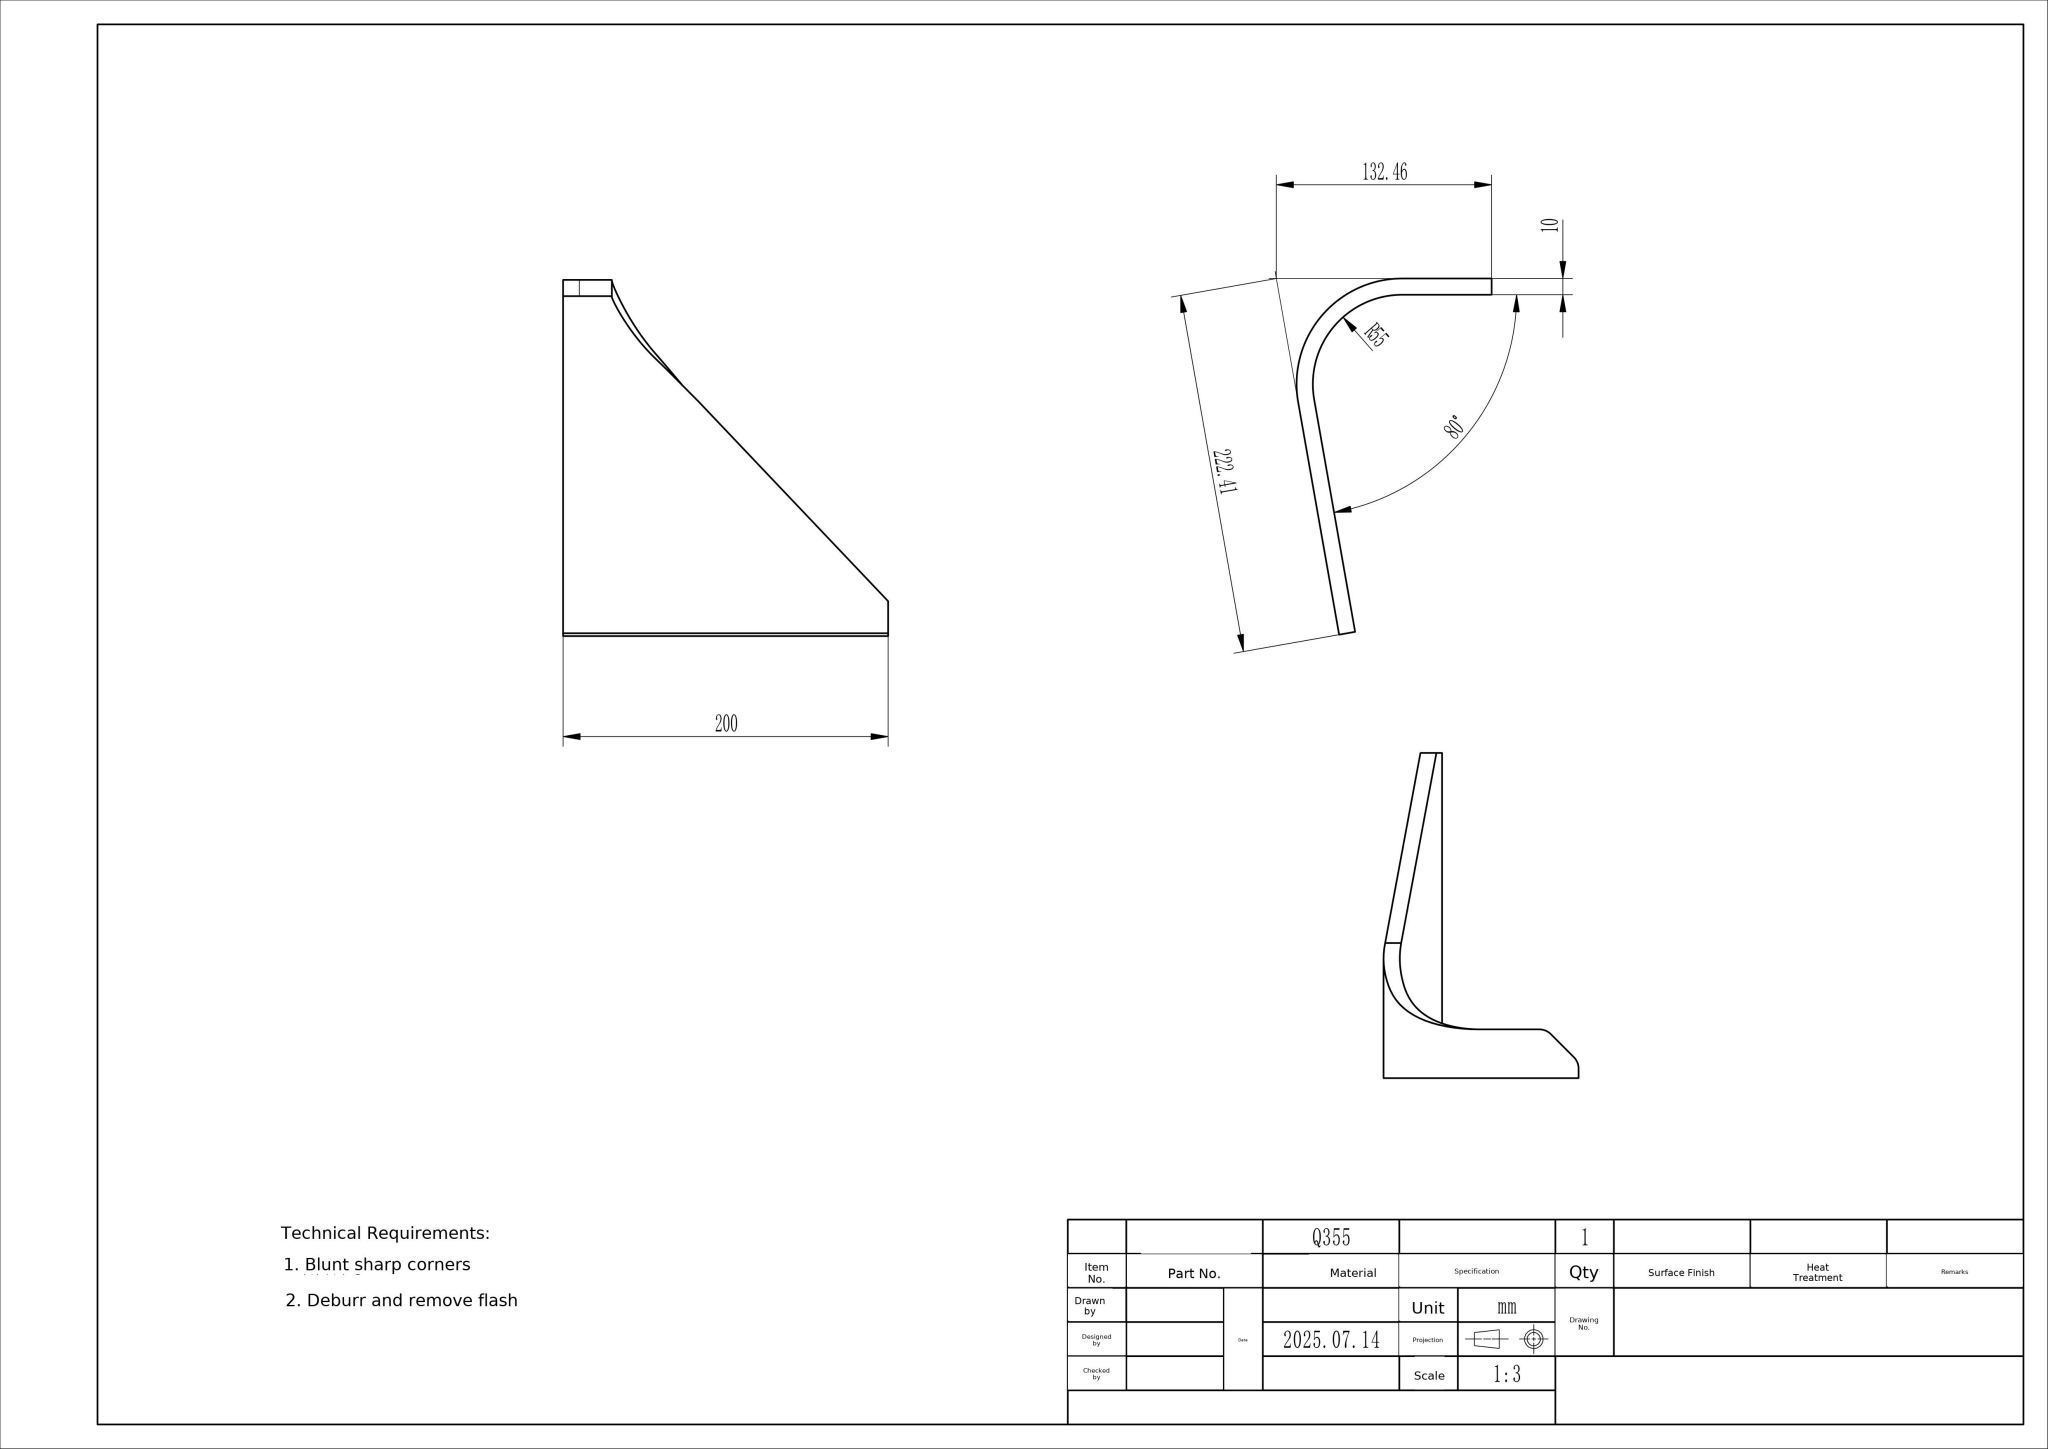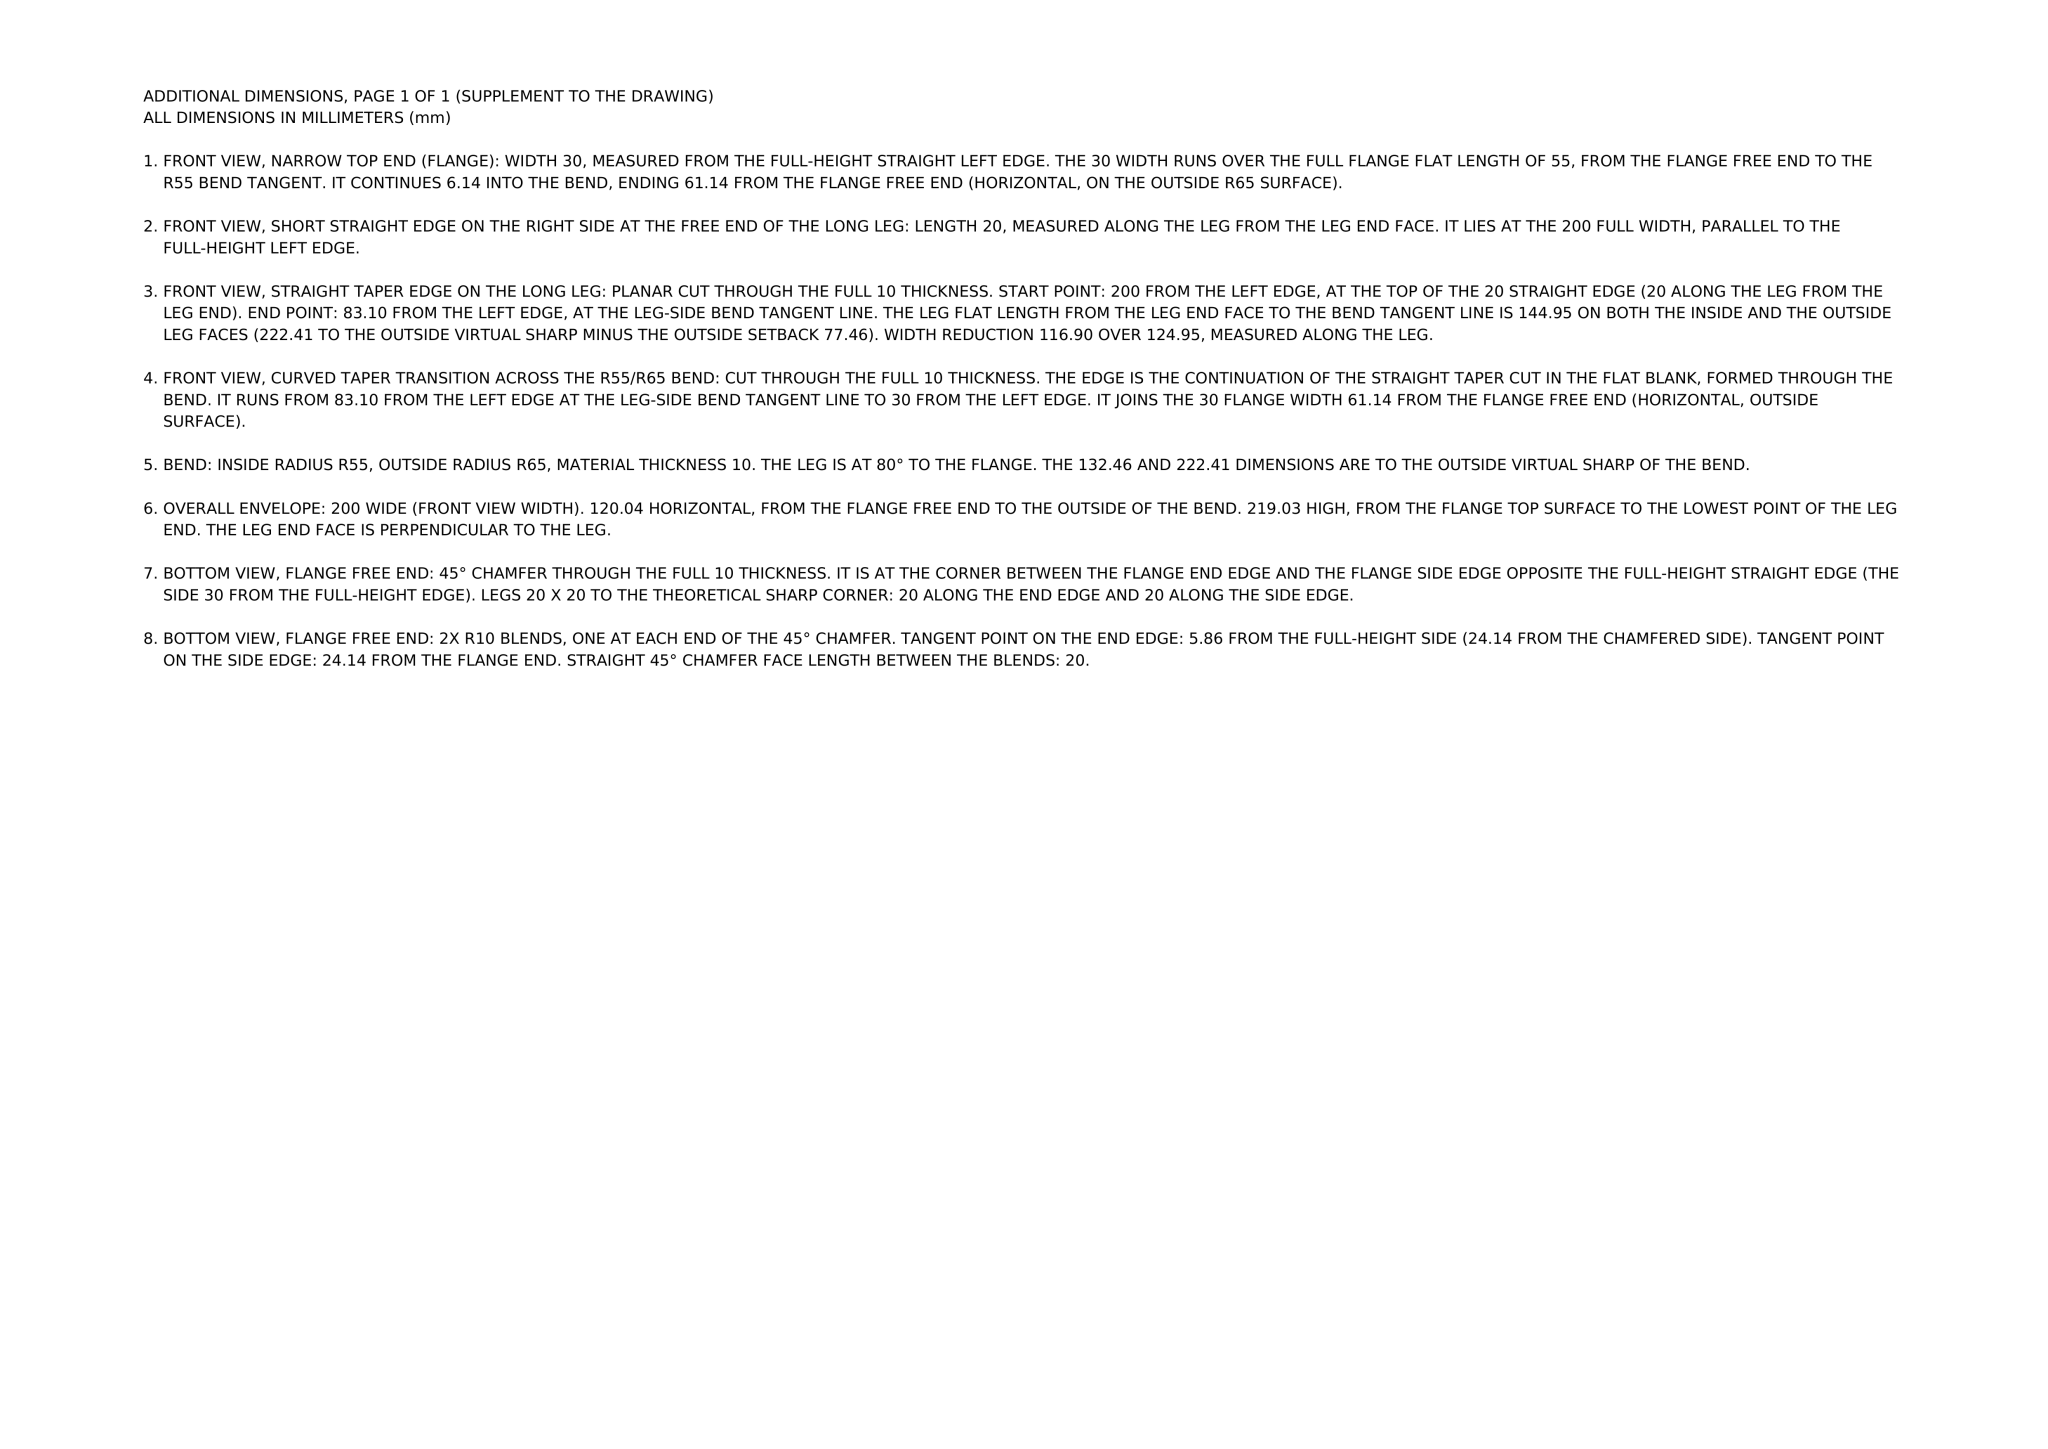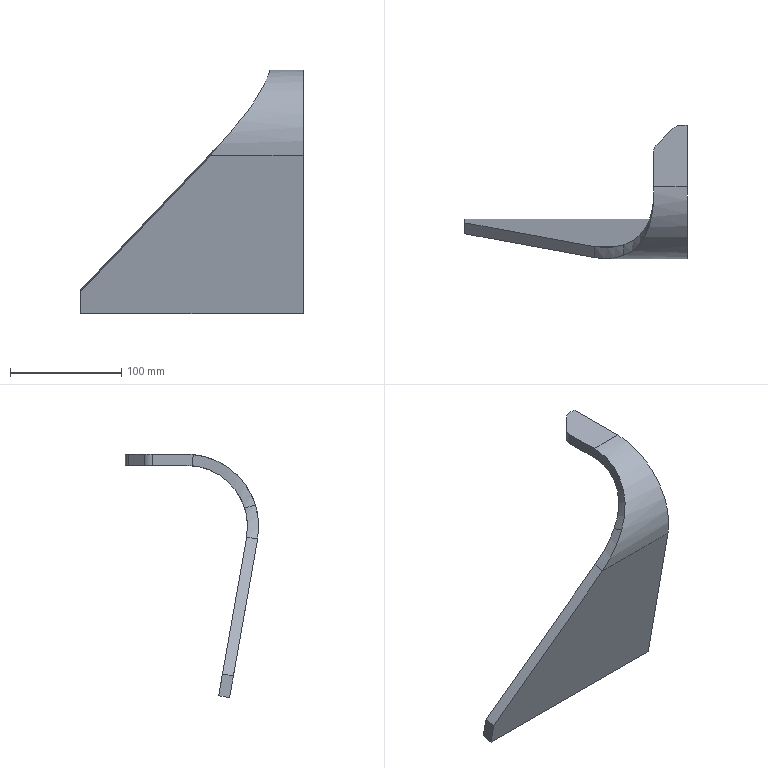Part | NX | mm | 1 solid | 17 faces | box 200 x 120 x 219.03 mm | volume 280175 mm3 | plane 11 | cylinder 4 | spline 2 | commonest cylinder face diameters 20 x2 130 x1 110 x1
STEP:
#1=CARTESIAN_POINT('',(0.,0.,0.));
#2=DIRECTION('',(0.,0.,1.));
#3=DIRECTION('',(1.,0.,0.));
#4=AXIS2_PLACEMENT_3D('',#1,#2,#3);
#5=(LENGTH_UNIT()NAMED_UNIT(*)SI_UNIT(.MILLI.,.METRE.));
#6=UNCERTAINTY_MEASURE_WITH_UNIT(LENGTH_MEASURE(0.0508),#5,'','');
#7=(NAMED_UNIT(*)PLANE_ANGLE_UNIT()SI_UNIT($,.RADIAN.));
#8=PLANE_ANGLE_MEASURE_WITH_UNIT(PLANE_ANGLE_MEASURE(0.01745),#7);
#9=DIMENSIONAL_EXPONENTS(0.,0.,0.,0.,0.,0.,0.);
#10=(CONVERSION_BASED_UNIT('',#8)NAMED_UNIT(#9)PLANE_ANGLE_UNIT());
#11=(NAMED_UNIT(*)SI_UNIT($,.STERADIAN.)SOLID_ANGLE_UNIT());
#12=(GEOMETRIC_REPRESENTATION_CONTEXT(3)GLOBAL_UNCERTAINTY_ASSIGNED_CONTEXT((#6))GLOBAL_UNIT_ASSIGNED_CONTEXT((#5,#10,#11))REPRESENTATION_CONTEXT('',''));
#13=SHAPE_REPRESENTATION('',(#4),#12);
#14=CARTESIAN_POINT('',(0.,-83.995,-207.296));
#15=VERTEX_POINT('',#14);
#16=CARTESIAN_POINT('',(0.,-109.164,-64.551));
#17=VERTEX_POINT('',#16);
#18=CARTESIAN_POINT('',(0.,-119.019,-8.66));
#19=DIRECTION('',(-0.,-0.1736,0.9848));
#20=VECTOR('',#19,1.);
#21=LINE('',#18,#20);
#22=EDGE_CURVE('',#15,#17,#21,.T.);
#23=ORIENTED_EDGE('',*,*,#22,.T.);
#24=CARTESIAN_POINT('',(-0.,-55.,0.));
#25=VERTEX_POINT('',#24);
#26=CARTESIAN_POINT('',(0.,-55.,-55.));
#27=DIRECTION('',(-1.,0.,0.));
#28=DIRECTION('',(0.,0.,-1.));
#29=AXIS2_PLACEMENT_3D('',#26,#27,#28);
#30=CIRCLE('',#29,55.);
#31=EDGE_CURVE('',#17,#25,#30,.T.);
#32=ORIENTED_EDGE('',*,*,#31,.T.);
#33=CARTESIAN_POINT('',(0.,0.,0.));
#34=VERTEX_POINT('',#33);
#35=CARTESIAN_POINT('',(0.,-100.,0.));
#36=DIRECTION('',(-0.,1.,0.));
#37=VECTOR('',#36,1.);
#38=LINE('',#35,#37);
#39=EDGE_CURVE('',#25,#34,#38,.T.);
#40=ORIENTED_EDGE('',*,*,#39,.T.);
#41=CARTESIAN_POINT('',(0.,0.,10.));
#42=VERTEX_POINT('',#41);
#43=CARTESIAN_POINT('',(0.,0.,10.));
#44=DIRECTION('',(0.,0.,1.));
#45=VECTOR('',#44,1.);
#46=LINE('',#43,#45);
#47=EDGE_CURVE('',#34,#42,#46,.T.);
#48=ORIENTED_EDGE('',*,*,#47,.T.);
#49=CARTESIAN_POINT('',(0.,-55.,10.));
#50=VERTEX_POINT('',#49);
#51=CARTESIAN_POINT('',(0.,0.,10.));
#52=DIRECTION('',(-0.,1.,0.));
#53=VECTOR('',#52,1.);
#54=LINE('',#51,#53);
#55=EDGE_CURVE('',#50,#42,#54,.T.);
#56=ORIENTED_EDGE('',*,*,#55,.F.);
#57=CARTESIAN_POINT('',(0.,-119.013,-66.287));
#58=VERTEX_POINT('',#57);
#59=CARTESIAN_POINT('',(0.,-55.,-55.));
#60=DIRECTION('',(-1.,0.,0.));
#61=DIRECTION('',(0.,0.,-1.));
#62=AXIS2_PLACEMENT_3D('',#59,#60,#61);
#63=CIRCLE('',#62,65.);
#64=EDGE_CURVE('',#58,#50,#63,.T.);
#65=ORIENTED_EDGE('',*,*,#64,.F.);
#66=CARTESIAN_POINT('',(0.,-93.843,-209.032));
#67=VERTEX_POINT('',#66);
#68=CARTESIAN_POINT('',(0.,-146.232,88.084));
#69=DIRECTION('',(-0.,-0.1736,0.9848));
#70=VECTOR('',#69,1.);
#71=LINE('',#68,#70);
#72=EDGE_CURVE('',#67,#58,#71,.T.);
#73=ORIENTED_EDGE('',*,*,#72,.F.);
#74=CARTESIAN_POINT('',(0.,-93.843,-209.032));
#75=DIRECTION('',(0.,-0.9848,-0.1736));
#76=VECTOR('',#75,1.);
#77=LINE('',#74,#76);
#78=EDGE_CURVE('',#15,#67,#77,.T.);
#79=ORIENTED_EDGE('',*,*,#78,.F.);
#80=EDGE_LOOP('',(#23,#32,#40,#48,#56,#65,#73,#79));
#81=FACE_OUTER_BOUND('',#80,.T.);
#82=CARTESIAN_POINT('',(0.,-128.868,-10.397));
#83=DIRECTION('',(1.,-0.,0.));
#84=DIRECTION('',(-0.,-0.1736,0.9848));
#85=AXIS2_PLACEMENT_3D('',#82,#83,#84);
#86=PLANE('',#85);
#87=ADVANCED_FACE('',(#81),#86,.T.);
#88=CARTESIAN_POINT('',(-200.,-87.468,-187.6));
#89=VERTEX_POINT('',#88);
#90=CARTESIAN_POINT('',(-83.098,-109.164,-64.551));
#91=VERTEX_POINT('',#90);
#92=CARTESIAN_POINT('',(-200.,-87.468,-187.6));
#93=DIRECTION('',(0.6832,-0.1268,0.7191));
#94=VECTOR('',#93,1.);
#95=LINE('',#92,#94);
#96=EDGE_CURVE('',#89,#91,#95,.T.);
#97=ORIENTED_EDGE('',*,*,#96,.T.);
#98=CARTESIAN_POINT('',(-290.,-109.164,-64.551));
#99=DIRECTION('',(1.,0.,0.));
#100=VECTOR('',#99,1.);
#101=LINE('',#98,#100);
#102=EDGE_CURVE('',#91,#17,#101,.T.);
#103=ORIENTED_EDGE('',*,*,#102,.T.);
#104=ORIENTED_EDGE('',*,*,#22,.F.);
#105=CARTESIAN_POINT('',(-200.,-83.995,-207.296));
#106=VERTEX_POINT('',#105);
#107=CARTESIAN_POINT('',(0.,-83.995,-207.296));
#108=DIRECTION('',(1.,-0.,0.));
#109=VECTOR('',#108,1.);
#110=LINE('',#107,#109);
#111=EDGE_CURVE('',#106,#15,#110,.T.);
#112=ORIENTED_EDGE('',*,*,#111,.F.);
#113=CARTESIAN_POINT('',(-200.,-83.995,-207.296));
#114=DIRECTION('',(0.,-0.1736,0.9848));
#115=VECTOR('',#114,1.);
#116=LINE('',#113,#115);
#117=EDGE_CURVE('',#106,#89,#116,.T.);
#118=ORIENTED_EDGE('',*,*,#117,.T.);
#119=EDGE_LOOP('',(#97,#103,#104,#112,#118));
#120=FACE_OUTER_BOUND('',#119,.T.);
#121=CARTESIAN_POINT('',(-130.,-125.876,30.226));
#122=DIRECTION('',(0.,-0.9848,-0.1736));
#123=DIRECTION('',(1.,0.,0.));
#124=AXIS2_PLACEMENT_3D('',#121,#122,#123);
#125=PLANE('',#124);
#126=ADVANCED_FACE('',(#120),#125,.F.);
#127=ORIENTED_EDGE('',*,*,#111,.T.);
#128=ORIENTED_EDGE('',*,*,#78,.T.);
#129=CARTESIAN_POINT('',(-200.,-93.843,-209.032));
#130=VERTEX_POINT('',#129);
#131=CARTESIAN_POINT('',(0.,-93.843,-209.032));
#132=DIRECTION('',(1.,-0.,0.));
#133=VECTOR('',#132,1.);
#134=LINE('',#131,#133);
#135=EDGE_CURVE('',#130,#67,#134,.T.);
#136=ORIENTED_EDGE('',*,*,#135,.F.);
#137=CARTESIAN_POINT('',(-200.,-93.843,-209.032));
#138=DIRECTION('',(0.,0.9848,0.1736));
#139=VECTOR('',#138,1.);
#140=LINE('',#137,#139);
#141=EDGE_CURVE('',#130,#106,#140,.T.);
#142=ORIENTED_EDGE('',*,*,#141,.T.);
#143=EDGE_LOOP('',(#127,#128,#136,#142));
#144=FACE_OUTER_BOUND('',#143,.T.);
#145=CARTESIAN_POINT('',(0.,-93.843,-209.032));
#146=DIRECTION('',(0.,0.1736,-0.9848));
#147=DIRECTION('',(1.,-0.,0.));
#148=AXIS2_PLACEMENT_3D('',#145,#146,#147);
#149=PLANE('',#148);
#150=ADVANCED_FACE('',(#144),#149,.T.);
#151=ORIENTED_EDGE('',*,*,#117,.F.);
#152=ORIENTED_EDGE('',*,*,#141,.F.);
#153=CARTESIAN_POINT('',(-200.,-97.316,-189.336));
#154=VERTEX_POINT('',#153);
#155=CARTESIAN_POINT('',(-200.,-93.843,-209.032));
#156=DIRECTION('',(0.,-0.1736,0.9848));
#157=VECTOR('',#156,1.);
#158=LINE('',#155,#157);
#159=EDGE_CURVE('',#130,#154,#158,.T.);
#160=ORIENTED_EDGE('',*,*,#159,.T.);
#161=CARTESIAN_POINT('',(-200.,-97.316,-189.336));
#162=DIRECTION('',(0.,0.9848,0.1736));
#163=VECTOR('',#162,1.);
#164=LINE('',#161,#163);
#165=EDGE_CURVE('',#154,#89,#164,.T.);
#166=ORIENTED_EDGE('',*,*,#165,.T.);
#167=EDGE_LOOP('',(#151,#152,#160,#166));
#168=FACE_OUTER_BOUND('',#167,.T.);
#169=CARTESIAN_POINT('',(-200.,-93.843,-209.032));
#170=DIRECTION('',(-1.,0.,0.));
#171=DIRECTION('',(0.,-0.9848,-0.1736));
#172=AXIS2_PLACEMENT_3D('',#169,#170,#171);
#173=PLANE('',#172);
#174=ADVANCED_FACE('',(#168),#173,.T.);
#175=CARTESIAN_POINT('',(-83.098,-119.013,-66.287));
#176=VERTEX_POINT('',#175);
#177=CARTESIAN_POINT('',(-83.098,-119.013,-66.287));
#178=DIRECTION('',(-0.,-0.9848,-0.1736));
#179=VECTOR('',#178,1.);
#180=LINE('',#177,#179);
#181=EDGE_CURVE('',#91,#176,#180,.T.);
#182=ORIENTED_EDGE('',*,*,#181,.F.);
#183=ORIENTED_EDGE('',*,*,#96,.F.);
#184=ORIENTED_EDGE('',*,*,#165,.F.);
#185=CARTESIAN_POINT('',(-200.,-97.316,-189.336));
#186=DIRECTION('',(0.6832,-0.1268,0.7191));
#187=VECTOR('',#186,1.);
#188=LINE('',#185,#187);
#189=EDGE_CURVE('',#154,#176,#188,.T.);
#190=ORIENTED_EDGE('',*,*,#189,.T.);
#191=EDGE_LOOP('',(#182,#183,#184,#190));
#192=FACE_OUTER_BOUND('',#191,.T.);
#193=CARTESIAN_POINT('',(-200.,-97.316,-189.336));
#194=DIRECTION('',(-0.7302,-0.1186,0.6728));
#195=DIRECTION('',(-0.6832,0.1268,-0.7191));
#196=AXIS2_PLACEMENT_3D('',#193,#194,#195);
#197=PLANE('',#196);
#198=ADVANCED_FACE('',(#192),#197,.T.);
#199=CARTESIAN_POINT('',(-290.,-119.013,-66.287));
#200=DIRECTION('',(1.,0.,0.));
#201=VECTOR('',#200,1.);
#202=LINE('',#199,#201);
#203=EDGE_CURVE('',#176,#58,#202,.T.);
#204=ORIENTED_EDGE('',*,*,#203,.F.);
#205=ORIENTED_EDGE('',*,*,#189,.F.);
#206=ORIENTED_EDGE('',*,*,#159,.F.);
#207=ORIENTED_EDGE('',*,*,#135,.T.);
#208=ORIENTED_EDGE('',*,*,#72,.T.);
#209=EDGE_LOOP('',(#204,#205,#206,#207,#208));
#210=FACE_OUTER_BOUND('',#209,.T.);
#211=CARTESIAN_POINT('',(-130.,-135.724,28.49));
#212=DIRECTION('',(0.,-0.9848,-0.1736));
#213=DIRECTION('',(1.,0.,0.));
#214=AXIS2_PLACEMENT_3D('',#211,#212,#213);
#215=PLANE('',#214);
#216=ADVANCED_FACE('',(#210),#215,.T.);
#217=CARTESIAN_POINT('',(-5.858,-0.,0.));
#218=VERTEX_POINT('',#217);
#219=CARTESIAN_POINT('',(-10.,-0.,0.));
#220=DIRECTION('',(-1.,-0.,0.));
#221=VECTOR('',#220,1.);
#222=LINE('',#219,#221);
#223=EDGE_CURVE('',#34,#218,#222,.T.);
#224=ORIENTED_EDGE('',*,*,#223,.T.);
#225=CARTESIAN_POINT('',(-5.858,-0.,10.));
#226=VERTEX_POINT('',#225);
#227=CARTESIAN_POINT('',(-5.858,-0.,10.));
#228=DIRECTION('',(0.,0.,1.));
#229=VECTOR('',#228,1.);
#230=LINE('',#227,#229);
#231=EDGE_CURVE('',#218,#226,#230,.T.);
#232=ORIENTED_EDGE('',*,*,#231,.T.);
#233=CARTESIAN_POINT('',(-10.,-0.,10.));
#234=DIRECTION('',(-1.,-0.,0.));
#235=VECTOR('',#234,1.);
#236=LINE('',#233,#235);
#237=EDGE_CURVE('',#42,#226,#236,.T.);
#238=ORIENTED_EDGE('',*,*,#237,.F.);
#239=ORIENTED_EDGE('',*,*,#47,.F.);
#240=EDGE_LOOP('',(#224,#232,#238,#239));
#241=FACE_OUTER_BOUND('',#240,.T.);
#242=CARTESIAN_POINT('',(-10.,-0.,10.));
#243=DIRECTION('',(-0.,1.,0.));
#244=DIRECTION('',(-1.,-0.,0.));
#245=AXIS2_PLACEMENT_3D('',#242,#243,#244);
#246=PLANE('',#245);
#247=ADVANCED_FACE('',(#241),#246,.T.);
#248=CARTESIAN_POINT('',(-27.071,-17.071,10.));
#249=VERTEX_POINT('',#248);
#250=CARTESIAN_POINT('',(-12.929,-2.929,10.));
#251=VERTEX_POINT('',#250);
#252=CARTESIAN_POINT('',(-30.,-20.,10.));
#253=DIRECTION('',(0.7071,0.7071,0.));
#254=VECTOR('',#253,1.);
#255=LINE('',#252,#254);
#256=EDGE_CURVE('',#249,#251,#255,.T.);
#257=ORIENTED_EDGE('',*,*,#256,.T.);
#258=CARTESIAN_POINT('',(-12.929,-2.929,0.));
#259=VERTEX_POINT('',#258);
#260=CARTESIAN_POINT('',(-12.929,-2.929,10.));
#261=DIRECTION('',(0.,0.,-1.));
#262=VECTOR('',#261,1.);
#263=LINE('',#260,#262);
#264=EDGE_CURVE('',#251,#259,#263,.T.);
#265=ORIENTED_EDGE('',*,*,#264,.T.);
#266=CARTESIAN_POINT('',(-27.071,-17.071,0.));
#267=VERTEX_POINT('',#266);
#268=CARTESIAN_POINT('',(-30.,-20.,0.));
#269=DIRECTION('',(0.7071,0.7071,0.));
#270=VECTOR('',#269,1.);
#271=LINE('',#268,#270);
#272=EDGE_CURVE('',#267,#259,#271,.T.);
#273=ORIENTED_EDGE('',*,*,#272,.F.);
#274=CARTESIAN_POINT('',(-27.071,-17.071,10.));
#275=DIRECTION('',(0.,0.,1.));
#276=VECTOR('',#275,1.);
#277=LINE('',#274,#276);
#278=EDGE_CURVE('',#267,#249,#277,.T.);
#279=ORIENTED_EDGE('',*,*,#278,.T.);
#280=EDGE_LOOP('',(#257,#265,#273,#279));
#281=FACE_OUTER_BOUND('',#280,.T.);
#282=CARTESIAN_POINT('',(-30.,-20.,10.));
#283=DIRECTION('',(-0.7071,0.7071,0.));
#284=DIRECTION('',(-0.7071,-0.7071,0.));
#285=AXIS2_PLACEMENT_3D('',#282,#283,#284);
#286=PLANE('',#285);
#287=ADVANCED_FACE('',(#281),#286,.T.);
#288=ORIENTED_EDGE('',*,*,#272,.T.);
#289=CARTESIAN_POINT('',(-5.858,-10.,0.));
#290=DIRECTION('',(0.,0.,-1.));
#291=DIRECTION('',(1.,0.,0.));
#292=AXIS2_PLACEMENT_3D('',#289,#290,#291);
#293=CIRCLE('',#292,10.);
#294=EDGE_CURVE('',#259,#218,#293,.T.);
#295=ORIENTED_EDGE('',*,*,#294,.T.);
#296=ORIENTED_EDGE('',*,*,#223,.F.);
#297=ORIENTED_EDGE('',*,*,#39,.F.);
#298=CARTESIAN_POINT('',(-30.,-55.,0.));
#299=VERTEX_POINT('',#298);
#300=CARTESIAN_POINT('',(-290.,-55.,0.));
#301=DIRECTION('',(-1.,0.,0.));
#302=VECTOR('',#301,1.);
#303=LINE('',#300,#302);
#304=EDGE_CURVE('',#25,#299,#303,.T.);
#305=ORIENTED_EDGE('',*,*,#304,.T.);
#306=CARTESIAN_POINT('',(-30.,-24.142,0.));
#307=VERTEX_POINT('',#306);
#308=CARTESIAN_POINT('',(-30.,-60.514,0.));
#309=DIRECTION('',(0.,-1.,0.));
#310=VECTOR('',#309,1.);
#311=LINE('',#308,#310);
#312=EDGE_CURVE('',#307,#299,#311,.T.);
#313=ORIENTED_EDGE('',*,*,#312,.F.);
#314=CARTESIAN_POINT('',(-20.,-24.142,0.));
#315=DIRECTION('',(0.,0.,-1.));
#316=DIRECTION('',(1.,0.,0.));
#317=AXIS2_PLACEMENT_3D('',#314,#315,#316);
#318=CIRCLE('',#317,10.);
#319=EDGE_CURVE('',#307,#267,#318,.T.);
#320=ORIENTED_EDGE('',*,*,#319,.T.);
#321=EDGE_LOOP('',(#288,#295,#296,#297,#305,#313,#320));
#322=FACE_OUTER_BOUND('',#321,.T.);
#323=CARTESIAN_POINT('',(-130.,-60.514,0.));
#324=DIRECTION('',(0.,0.,1.));
#325=DIRECTION('',(1.,0.,0.));
#326=AXIS2_PLACEMENT_3D('',#323,#324,#325);
#327=PLANE('',#326);
#328=ADVANCED_FACE('',(#322),#327,.F.);
#329=CARTESIAN_POINT('',(-30.,-24.142,10.));
#330=VERTEX_POINT('',#329);
#331=CARTESIAN_POINT('',(-30.,-55.,10.));
#332=VERTEX_POINT('',#331);
#333=CARTESIAN_POINT('',(-30.,-60.514,10.));
#334=DIRECTION('',(0.,-1.,0.));
#335=VECTOR('',#334,1.);
#336=LINE('',#333,#335);
#337=EDGE_CURVE('',#330,#332,#336,.T.);
#338=ORIENTED_EDGE('',*,*,#337,.F.);
#339=CARTESIAN_POINT('',(-30.,-24.142,10.));
#340=DIRECTION('',(0.,0.,-1.));
#341=VECTOR('',#340,1.);
#342=LINE('',#339,#341);
#343=EDGE_CURVE('',#330,#307,#342,.T.);
#344=ORIENTED_EDGE('',*,*,#343,.T.);
#345=ORIENTED_EDGE('',*,*,#312,.T.);
#346=CARTESIAN_POINT('',(-30.,-60.194,-0.2458));
#347=VERTEX_POINT('',#346);
#348=CARTESIAN_POINT('',(-30.,-55.,-55.));
#349=DIRECTION('',(1.,0.,0.));
#350=DIRECTION('',(0.,0.,-1.));
#351=AXIS2_PLACEMENT_3D('',#348,#349,#350);
#352=CIRCLE('',#351,55.);
#353=EDGE_CURVE('',#299,#347,#352,.T.);
#354=ORIENTED_EDGE('',*,*,#353,.T.);
#355=CARTESIAN_POINT('',(-30.,-61.138,9.71));
#356=VERTEX_POINT('',#355);
#357=CARTESIAN_POINT('',(-30.,-60.194,-0.2458));
#358=DIRECTION('',(0.,-0.09443,0.9955));
#359=VECTOR('',#358,1.);
#360=LINE('',#357,#359);
#361=EDGE_CURVE('',#347,#356,#360,.T.);
#362=ORIENTED_EDGE('',*,*,#361,.T.);
#363=CARTESIAN_POINT('',(-30.,-55.,-55.));
#364=DIRECTION('',(1.,0.,0.));
#365=DIRECTION('',(0.,0.,-1.));
#366=AXIS2_PLACEMENT_3D('',#363,#364,#365);
#367=CIRCLE('',#366,65.);
#368=EDGE_CURVE('',#332,#356,#367,.T.);
#369=ORIENTED_EDGE('',*,*,#368,.F.);
#370=EDGE_LOOP('',(#338,#344,#345,#354,#362,#369));
#371=FACE_OUTER_BOUND('',#370,.T.);
#372=CARTESIAN_POINT('',(-30.,-60.514,10.));
#373=DIRECTION('',(-1.,-0.,0.));
#374=DIRECTION('',(0.,-1.,0.));
#375=AXIS2_PLACEMENT_3D('',#372,#373,#374);
#376=PLANE('',#375);
#377=ADVANCED_FACE('',(#371),#376,.T.);
#378=ORIENTED_EDGE('',*,*,#237,.T.);
#379=CARTESIAN_POINT('',(-5.858,-10.,10.));
#380=DIRECTION('',(0.,0.,1.));
#381=DIRECTION('',(1.,0.,0.));
#382=AXIS2_PLACEMENT_3D('',#379,#380,#381);
#383=CIRCLE('',#382,10.);
#384=EDGE_CURVE('',#226,#251,#383,.T.);
#385=ORIENTED_EDGE('',*,*,#384,.T.);
#386=ORIENTED_EDGE('',*,*,#256,.F.);
#387=CARTESIAN_POINT('',(-20.,-24.142,10.));
#388=DIRECTION('',(0.,0.,1.));
#389=DIRECTION('',(1.,0.,0.));
#390=AXIS2_PLACEMENT_3D('',#387,#388,#389);
#391=CIRCLE('',#390,10.);
#392=EDGE_CURVE('',#249,#330,#391,.T.);
#393=ORIENTED_EDGE('',*,*,#392,.T.);
#394=ORIENTED_EDGE('',*,*,#337,.T.);
#395=CARTESIAN_POINT('',(-290.,-55.,10.));
#396=DIRECTION('',(-1.,0.,0.));
#397=VECTOR('',#396,1.);
#398=LINE('',#395,#397);
#399=EDGE_CURVE('',#50,#332,#398,.T.);
#400=ORIENTED_EDGE('',*,*,#399,.F.);
#401=ORIENTED_EDGE('',*,*,#55,.T.);
#402=EDGE_LOOP('',(#378,#385,#386,#393,#394,#400,#401));
#403=FACE_OUTER_BOUND('',#402,.T.);
#404=CARTESIAN_POINT('',(-130.,-60.514,10.));
#405=DIRECTION('',(0.,0.,1.));
#406=DIRECTION('',(1.,0.,0.));
#407=AXIS2_PLACEMENT_3D('',#404,#405,#406);
#408=PLANE('',#407);
#409=ADVANCED_FACE('',(#403),#408,.T.);
#410=ORIENTED_EDGE('',*,*,#361,.F.);
#411=CARTESIAN_POINT('',(-56.977,-107.472,-38.518));
#412=VERTEX_POINT('',#411);
#413=CARTESIAN_POINT('',(-56.977,-107.472,-38.518));
#414=CARTESIAN_POINT('',(-52.695,-106.178,-34.399));
#415=CARTESIAN_POINT('',(-48.845,-104.275,-30.061));
#416=CARTESIAN_POINT('',(-42.142,-98.974,-21.589));
#417=CARTESIAN_POINT('',(-39.291,-95.572,-17.461));
#418=CARTESIAN_POINT('',(-34.687,-87.335,-10.17));
#419=CARTESIAN_POINT('',(-32.934,-82.501,-7.016));
#420=CARTESIAN_POINT('',(-30.591,-71.871,-2.33));
#421=CARTESIAN_POINT('',(-30.,-66.08,-0.8041));
#422=CARTESIAN_POINT('',(-30.,-60.194,-0.2458));
#423=B_SPLINE_CURVE_WITH_KNOTS('',3,(#413,#414,#415,#416,#417,#418,#419,#420,#421,#422),.UNSPECIFIED.,.F.,.F.,(4,2,2,2,4),(0.,0.25,0.5,0.75,1.),.UNSPECIFIED.);
#424=EDGE_CURVE('',#412,#347,#423,.T.);
#425=ORIENTED_EDGE('',*,*,#424,.F.);
#426=CARTESIAN_POINT('',(-56.977,-117.013,-35.522));
#427=VERTEX_POINT('',#426);
#428=CARTESIAN_POINT('',(-56.977,-112.243,-37.02));
#429=DIRECTION('',(0.,-0.954,0.2997));
#430=VECTOR('',#429,1.);
#431=LINE('',#428,#430);
#432=EDGE_CURVE('',#412,#427,#431,.T.);
#433=ORIENTED_EDGE('',*,*,#432,.T.);
#434=CARTESIAN_POINT('',(-56.977,-117.013,-35.522));
#435=CARTESIAN_POINT('',(-54.836,-116.248,-33.087));
#436=CARTESIAN_POINT('',(-52.803,-115.306,-30.59));
#437=CARTESIAN_POINT('',(-48.969,-113.016,-25.558));
#438=CARTESIAN_POINT('',(-47.169,-111.668,-23.023));
#439=CARTESIAN_POINT('',(-43.818,-108.535,-18.017));
#440=CARTESIAN_POINT('',(-42.267,-106.75,-15.546));
#441=CARTESIAN_POINT('',(-39.428,-102.74,-10.778));
#442=CARTESIAN_POINT('',(-38.14,-100.515,-8.482));
#443=CARTESIAN_POINT('',(-35.838,-95.648,-4.174));
#444=CARTESIAN_POINT('',(-34.824,-93.006,-2.163));
#445=CARTESIAN_POINT('',(-33.079,-87.362,1.471));
#446=CARTESIAN_POINT('',(-32.348,-84.36,3.093));
#447=CARTESIAN_POINT('',(-31.177,-78.079,5.862));
#448=CARTESIAN_POINT('',(-30.736,-74.799,7.009));
#449=CARTESIAN_POINT('',(-30.148,-68.068,8.768));
#450=CARTESIAN_POINT('',(-30.,-64.617,9.38));
#451=CARTESIAN_POINT('',(-30.,-61.138,9.71));
#452=B_SPLINE_CURVE_WITH_KNOTS('',3,(#434,#435,#436,#437,#438,#439,#440,#441,#442,#443,#444,#445,#446,#447,#448,#449,#450,#451),.UNSPECIFIED.,.F.,.F.,(4,2,2,2,2,2,2,2,4),(0.,0.125,0.25,0.375,0.5,0.625,0.75,0.875,1.),.UNSPECIFIED.);
#453=EDGE_CURVE('',#427,#356,#452,.T.);
#454=ORIENTED_EDGE('',*,*,#453,.T.);
#455=EDGE_LOOP('',(#410,#425,#433,#454));
#456=FACE_OUTER_BOUND('',#455,.T.);
#457=CARTESIAN_POINT('',(-56.977,-117.013,-35.522));
#458=CARTESIAN_POINT('',(-54.836,-116.248,-33.087));
#459=CARTESIAN_POINT('',(-52.803,-115.306,-30.59));
#460=CARTESIAN_POINT('',(-48.969,-113.016,-25.558));
#461=CARTESIAN_POINT('',(-47.169,-111.668,-23.023));
#462=CARTESIAN_POINT('',(-43.818,-108.535,-18.017));
#463=CARTESIAN_POINT('',(-42.267,-106.75,-15.546));
#464=CARTESIAN_POINT('',(-39.428,-102.74,-10.778));
#465=CARTESIAN_POINT('',(-38.14,-100.515,-8.482));
#466=CARTESIAN_POINT('',(-35.838,-95.648,-4.174));
#467=CARTESIAN_POINT('',(-34.824,-93.006,-2.163));
#468=CARTESIAN_POINT('',(-33.079,-87.362,1.471));
#469=CARTESIAN_POINT('',(-32.348,-84.36,3.093));
#470=CARTESIAN_POINT('',(-31.177,-78.079,5.862));
#471=CARTESIAN_POINT('',(-30.736,-74.799,7.009));
#472=CARTESIAN_POINT('',(-30.148,-68.068,8.768));
#473=CARTESIAN_POINT('',(-30.,-64.617,9.38));
#474=CARTESIAN_POINT('',(-30.,-61.138,9.71));
#475=CARTESIAN_POINT('',(-56.977,-107.472,-38.518));
#476=CARTESIAN_POINT('',(-54.836,-106.825,-36.459));
#477=CARTESIAN_POINT('',(-52.803,-106.028,-34.346));
#478=CARTESIAN_POINT('',(-48.969,-104.09,-30.088));
#479=CARTESIAN_POINT('',(-47.169,-102.95,-27.943));
#480=CARTESIAN_POINT('',(-43.818,-100.299,-23.707));
#481=CARTESIAN_POINT('',(-42.267,-98.789,-21.616));
#482=CARTESIAN_POINT('',(-39.428,-95.396,-17.582));
#483=CARTESIAN_POINT('',(-38.14,-93.513,-15.638));
#484=CARTESIAN_POINT('',(-35.838,-89.394,-11.993));
#485=CARTESIAN_POINT('',(-34.824,-87.159,-10.291));
#486=CARTESIAN_POINT('',(-33.079,-82.384,-7.217));
#487=CARTESIAN_POINT('',(-32.348,-79.843,-5.845));
#488=CARTESIAN_POINT('',(-31.177,-74.528,-3.502));
#489=CARTESIAN_POINT('',(-30.736,-71.753,-2.531));
#490=CARTESIAN_POINT('',(-30.148,-66.058,-1.043));
#491=CARTESIAN_POINT('',(-30.,-63.137,-0.525));
#492=CARTESIAN_POINT('',(-30.,-60.194,-0.2458));
#493=B_SPLINE_SURFACE_WITH_KNOTS('',1,3,((#457,#458,#459,#460,#461,#462,#463,#464,#465,#466,#467,#468,#469,#470,#471,#472,#473,#474),(#475,#476,#477,#478,#479,#480,#481,#482,#483,#484,#485,#486,#487,#488,#489,#490,#491,#492)),.UNSPECIFIED.,.F.,.F.,.F.,(2,2),(4,2,2,2,2,2,2,2,4),(0.,1.),(0.,0.125,0.25,0.375,0.5,0.625,0.75,0.875,1.),.UNSPECIFIED.);
#494=ADVANCED_FACE('',(#456),#493,.F.);
#495=CARTESIAN_POINT('',(-83.098,-109.164,-64.551));
#496=CARTESIAN_POINT('',(-74.391,-110.689,-55.905));
#497=CARTESIAN_POINT('',(-65.684,-110.103,-46.894));
#498=CARTESIAN_POINT('',(-56.977,-107.472,-38.518));
#499=B_SPLINE_CURVE_WITH_KNOTS('',3,(#495,#496,#497,#498),.UNSPECIFIED.,.F.,.F.,(4,4),(0.,1.),.UNSPECIFIED.);
#500=EDGE_CURVE('',#91,#412,#499,.T.);
#501=ORIENTED_EDGE('',*,*,#500,.F.);
#502=ORIENTED_EDGE('',*,*,#181,.T.);
#503=CARTESIAN_POINT('',(-83.098,-119.013,-66.287));
#504=CARTESIAN_POINT('',(-80.922,-119.463,-63.733));
#505=CARTESIAN_POINT('',(-78.745,-119.76,-61.151));
#506=CARTESIAN_POINT('',(-74.391,-120.044,-55.971));
#507=CARTESIAN_POINT('',(-72.215,-120.031,-53.373));
#508=CARTESIAN_POINT('',(-67.861,-119.695,-48.196));
#509=CARTESIAN_POINT('',(-65.684,-119.372,-45.617));
#510=CARTESIAN_POINT('',(-61.331,-118.419,-40.518));
#511=CARTESIAN_POINT('',(-59.154,-117.79,-37.996));
#512=CARTESIAN_POINT('',(-56.977,-117.013,-35.522));
#513=B_SPLINE_CURVE_WITH_KNOTS('',3,(#503,#504,#505,#506,#507,#508,#509,#510,#511,#512),.UNSPECIFIED.,.F.,.F.,(4,2,2,2,4),(0.,0.25,0.5,0.75,1.),.UNSPECIFIED.);
#514=EDGE_CURVE('',#176,#427,#513,.T.);
#515=ORIENTED_EDGE('',*,*,#514,.T.);
#516=ORIENTED_EDGE('',*,*,#432,.F.);
#517=EDGE_LOOP('',(#501,#502,#515,#516));
#518=FACE_OUTER_BOUND('',#517,.T.);
#519=CARTESIAN_POINT('',(-83.098,-119.013,-66.287));
#520=CARTESIAN_POINT('',(-80.922,-119.463,-63.733));
#521=CARTESIAN_POINT('',(-78.745,-119.76,-61.151));
#522=CARTESIAN_POINT('',(-74.391,-120.044,-55.971));
#523=CARTESIAN_POINT('',(-72.215,-120.031,-53.373));
#524=CARTESIAN_POINT('',(-67.861,-119.695,-48.196));
#525=CARTESIAN_POINT('',(-65.684,-119.372,-45.617));
#526=CARTESIAN_POINT('',(-61.331,-118.419,-40.518));
#527=CARTESIAN_POINT('',(-59.154,-117.79,-37.996));
#528=CARTESIAN_POINT('',(-56.977,-117.013,-35.522));
#529=CARTESIAN_POINT('',(-83.098,-109.164,-64.551));
#530=CARTESIAN_POINT('',(-80.922,-109.546,-62.389));
#531=CARTESIAN_POINT('',(-78.745,-109.797,-60.205));
#532=CARTESIAN_POINT('',(-74.391,-110.038,-55.822));
#533=CARTESIAN_POINT('',(-72.215,-110.027,-53.623));
#534=CARTESIAN_POINT('',(-67.861,-109.742,-49.242));
#535=CARTESIAN_POINT('',(-65.684,-109.468,-47.061));
#536=CARTESIAN_POINT('',(-61.331,-108.662,-42.746));
#537=CARTESIAN_POINT('',(-59.154,-108.13,-40.612));
#538=CARTESIAN_POINT('',(-56.977,-107.472,-38.518));
#539=B_SPLINE_SURFACE_WITH_KNOTS('',1,3,((#519,#520,#521,#522,#523,#524,#525,#526,#527,#528),(#529,#530,#531,#532,#533,#534,#535,#536,#537,#538)),.UNSPECIFIED.,.F.,.F.,.F.,(2,2),(4,2,2,2,4),(0.,1.),(0.,0.25,0.5,0.75,1.),.UNSPECIFIED.);
#540=ADVANCED_FACE('',(#518),#539,.F.);
#541=ORIENTED_EDGE('',*,*,#453,.F.);
#542=ORIENTED_EDGE('',*,*,#514,.F.);
#543=ORIENTED_EDGE('',*,*,#203,.T.);
#544=ORIENTED_EDGE('',*,*,#64,.T.);
#545=ORIENTED_EDGE('',*,*,#399,.T.);
#546=ORIENTED_EDGE('',*,*,#368,.T.);
#547=EDGE_LOOP('',(#541,#542,#543,#544,#545,#546));
#548=FACE_OUTER_BOUND('',#547,.T.);
#549=CARTESIAN_POINT('',(-30.,-55.,-55.));
#550=DIRECTION('',(1.,0.,0.));
#551=DIRECTION('',(0.,0.,-1.));
#552=AXIS2_PLACEMENT_3D('',#549,#550,#551);
#553=CYLINDRICAL_SURFACE('',#552,65.);
#554=ADVANCED_FACE('',(#548),#553,.T.);
#555=ORIENTED_EDGE('',*,*,#424,.T.);
#556=ORIENTED_EDGE('',*,*,#353,.F.);
#557=ORIENTED_EDGE('',*,*,#304,.F.);
#558=ORIENTED_EDGE('',*,*,#31,.F.);
#559=ORIENTED_EDGE('',*,*,#102,.F.);
#560=ORIENTED_EDGE('',*,*,#500,.T.);
#561=EDGE_LOOP('',(#555,#556,#557,#558,#559,#560));
#562=FACE_OUTER_BOUND('',#561,.T.);
#563=CARTESIAN_POINT('',(-30.,-55.,-55.));
#564=DIRECTION('',(1.,0.,0.));
#565=DIRECTION('',(0.,0.,-1.));
#566=AXIS2_PLACEMENT_3D('',#563,#564,#565);
#567=CYLINDRICAL_SURFACE('',#566,55.);
#568=ADVANCED_FACE('',(#562),#567,.F.);
#569=ORIENTED_EDGE('',*,*,#384,.F.);
#570=ORIENTED_EDGE('',*,*,#231,.F.);
#571=ORIENTED_EDGE('',*,*,#294,.F.);
#572=ORIENTED_EDGE('',*,*,#264,.F.);
#573=EDGE_LOOP('',(#569,#570,#571,#572));
#574=FACE_OUTER_BOUND('',#573,.T.);
#575=CARTESIAN_POINT('',(-5.858,-10.,10.));
#576=DIRECTION('',(0.,0.,-1.));
#577=DIRECTION('',(-1.,0.,0.));
#578=AXIS2_PLACEMENT_3D('',#575,#576,#577);
#579=CYLINDRICAL_SURFACE('',#578,10.);
#580=ADVANCED_FACE('',(#574),#579,.T.);
#581=ORIENTED_EDGE('',*,*,#392,.F.);
#582=ORIENTED_EDGE('',*,*,#278,.F.);
#583=ORIENTED_EDGE('',*,*,#319,.F.);
#584=ORIENTED_EDGE('',*,*,#343,.F.);
#585=EDGE_LOOP('',(#581,#582,#583,#584));
#586=FACE_OUTER_BOUND('',#585,.T.);
#587=CARTESIAN_POINT('',(-20.,-24.142,10.));
#588=DIRECTION('',(0.,0.,-1.));
#589=DIRECTION('',(-1.,0.,0.));
#590=AXIS2_PLACEMENT_3D('',#587,#588,#589);
#591=CYLINDRICAL_SURFACE('',#590,10.);
#592=ADVANCED_FACE('',(#586),#591,.T.);
#593=CLOSED_SHELL('',(#87,#126,#150,#174,#198,#216,#247,#287,#328,#377,#409,#494,#540,#554,#568,#580,#592));
#594=MANIFOLD_SOLID_BREP('',#593);
#595=ADVANCED_BREP_SHAPE_REPRESENTATION('',(#594),#12);
#596=SHAPE_REPRESENTATION_RELATIONSHIP('','',#13,#595);
#597=PRESENTATION_LAYER_ASSIGNMENT('','',(#594));
#598=COLOUR_RGB('',0.5961,0.6667,0.6863);
#599=FILL_AREA_STYLE_COLOUR('',#598);
#600=FILL_AREA_STYLE('',(#599));
#601=SURFACE_STYLE_FILL_AREA(#600);
#602=SURFACE_SIDE_STYLE('',(#601));
#603=SURFACE_STYLE_USAGE(.BOTH.,#602);
#604=PRESENTATION_STYLE_ASSIGNMENT((#603));
#605=STYLED_ITEM('',(#604),#594);
#606=MECHANICAL_DESIGN_GEOMETRIC_PRESENTATION_REPRESENTATION('',(#605),#12);